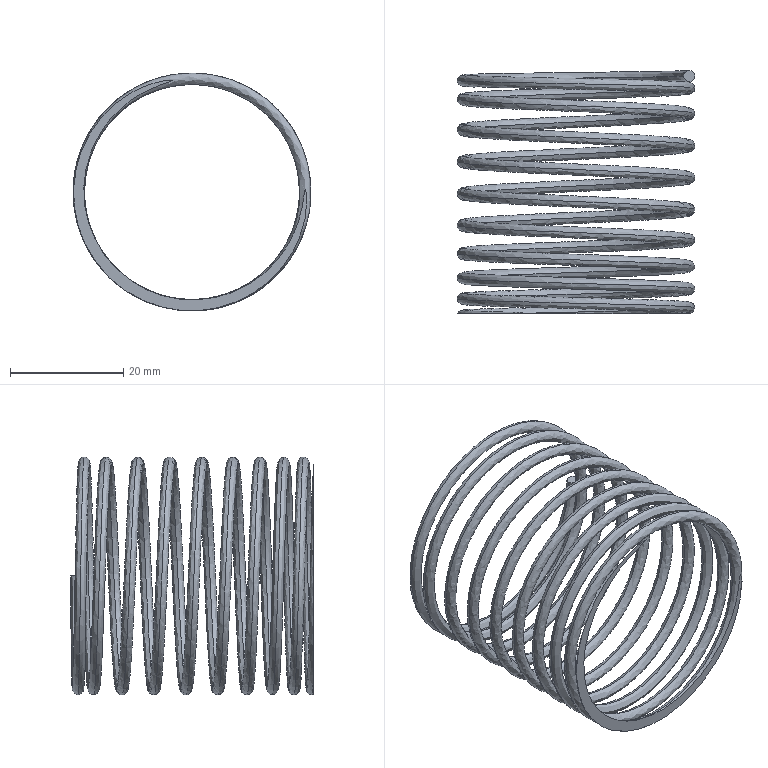Component | SolidWorks | spring3-1 | 1 solid | 4 faces | volume 3172 mm3 | spline 2 | plane 2